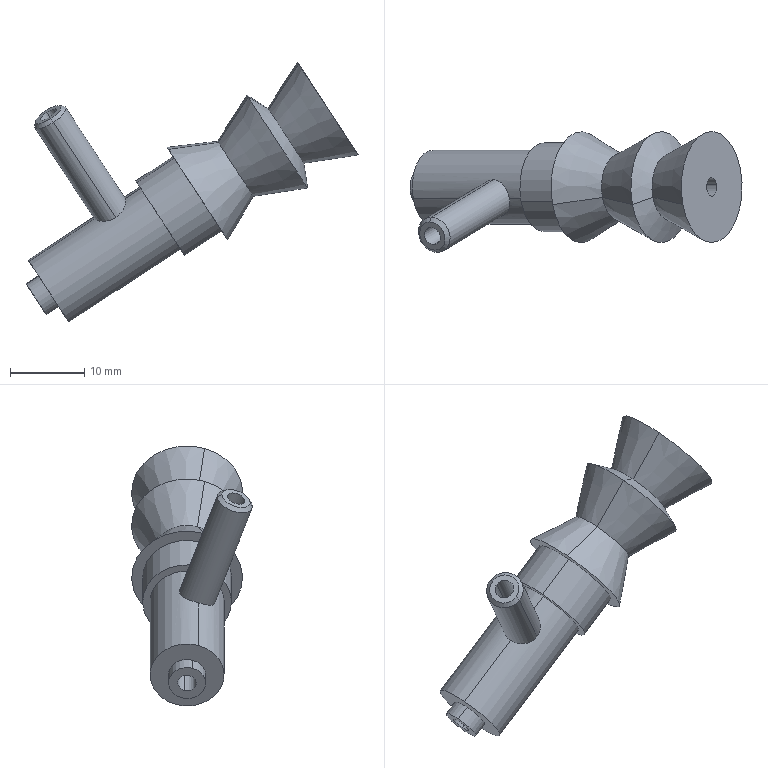Component | SolidWorks | SuctionCup3-1 | 1 solid | 37 faces | box 44.81 x 16.32 x 35.08 mm | volume 4543 mm3 | cylinder 19 | cone 10 | plane 8 | commonest cylinder face diameters 2.5 x7 5 x6 10 x4 12 x2
build123d program:
from build123d import *

# Parameters (mm, degrees)
SKETCH2_R               = 1.25
CUT_EXTRUDE1_DEPTH      = 59.962
CUT_EXTRUDE2_DEPTH      = 59.962
CUT_EXTRUDE2_DEPTH_BACK = 59.962
SKETCH3_W               = 23.814
SKETCH3_H               = 25.438
SKETCH4_R               = 2.5
SKETCH4_R_2             = 1.25
BOSS_EXTRUDE1_DEPTH     = 21
CHAMFER1_SIZE           = 0.5


with BuildPart() as part:
    # Sketch1 → Revolve1 (revolve)
    with BuildSketch(Plane.XY, mode=Mode.PRIVATE) as revolve1_sk:
        Polygon((0, 0), (2.5, 0), (2.5, -13), (5, -13), (5, -31), (6, -31), (6, -37), (7.489, -37), (4.431, -43.128), (7.5, -49.865), (4.431, -51.263), (7.5, -58), (0, -58), align=None)
    revolve(revolve1_sk.sketch.rotate(Axis((0, 0, 0), (0, -1, 0)), 90), axis=Axis((0, 0, 0), (0, -1, 0)))

    # Sketch2 → Cut-Extrude1 (cut, through all)
    with BuildSketch(Plane.XZ.offset(58)):
        with Locations(Location((0, 0, 0), (0, 0, 270))):
            Circle(SKETCH2_R)
    extrude(amount=-CUT_EXTRUDE1_DEPTH, mode=Mode.SUBTRACT)

    # Sketch3 → Cut-Extrude2 (cut, two sides: drawn at the far end of the back side and taken through both)
    with BuildSketch(Plane.XY.offset(-CUT_EXTRUDE2_DEPTH_BACK)):
        with Locations((1.119, 1.719)):
            Rectangle(SKETCH3_W, SKETCH3_H)
    extrude(amount=CUT_EXTRUDE2_DEPTH + CUT_EXTRUDE2_DEPTH_BACK, mode=Mode.SUBTRACT)

    # Sketch4 → Boss-Extrude1 (add)
    with BuildSketch(Plane.XY):
        with Locations(Location((0, -26, 0), (0, 0, 90))):
            Circle(SKETCH4_R)
        with Locations(Location((0, -26, 0), (0, 0, 270))):
            Circle(SKETCH4_R_2, mode=Mode.SUBTRACT)
    extrude(amount=BOSS_EXTRUDE1_DEPTH)

    # Chamfer1
    chamfer1_edges = [part.edges().sort_by_distance(p)[0] for p in [
        (0, -28.5, 21),
    ]]
    chamfer(chamfer1_edges, length=CHAMFER1_SIZE)


solid = part.part

# Placed as in the assembly
solid = solid.moved(Location((-250.899, -40.454, -149.126), (21.603, -31.283, 101.619)))